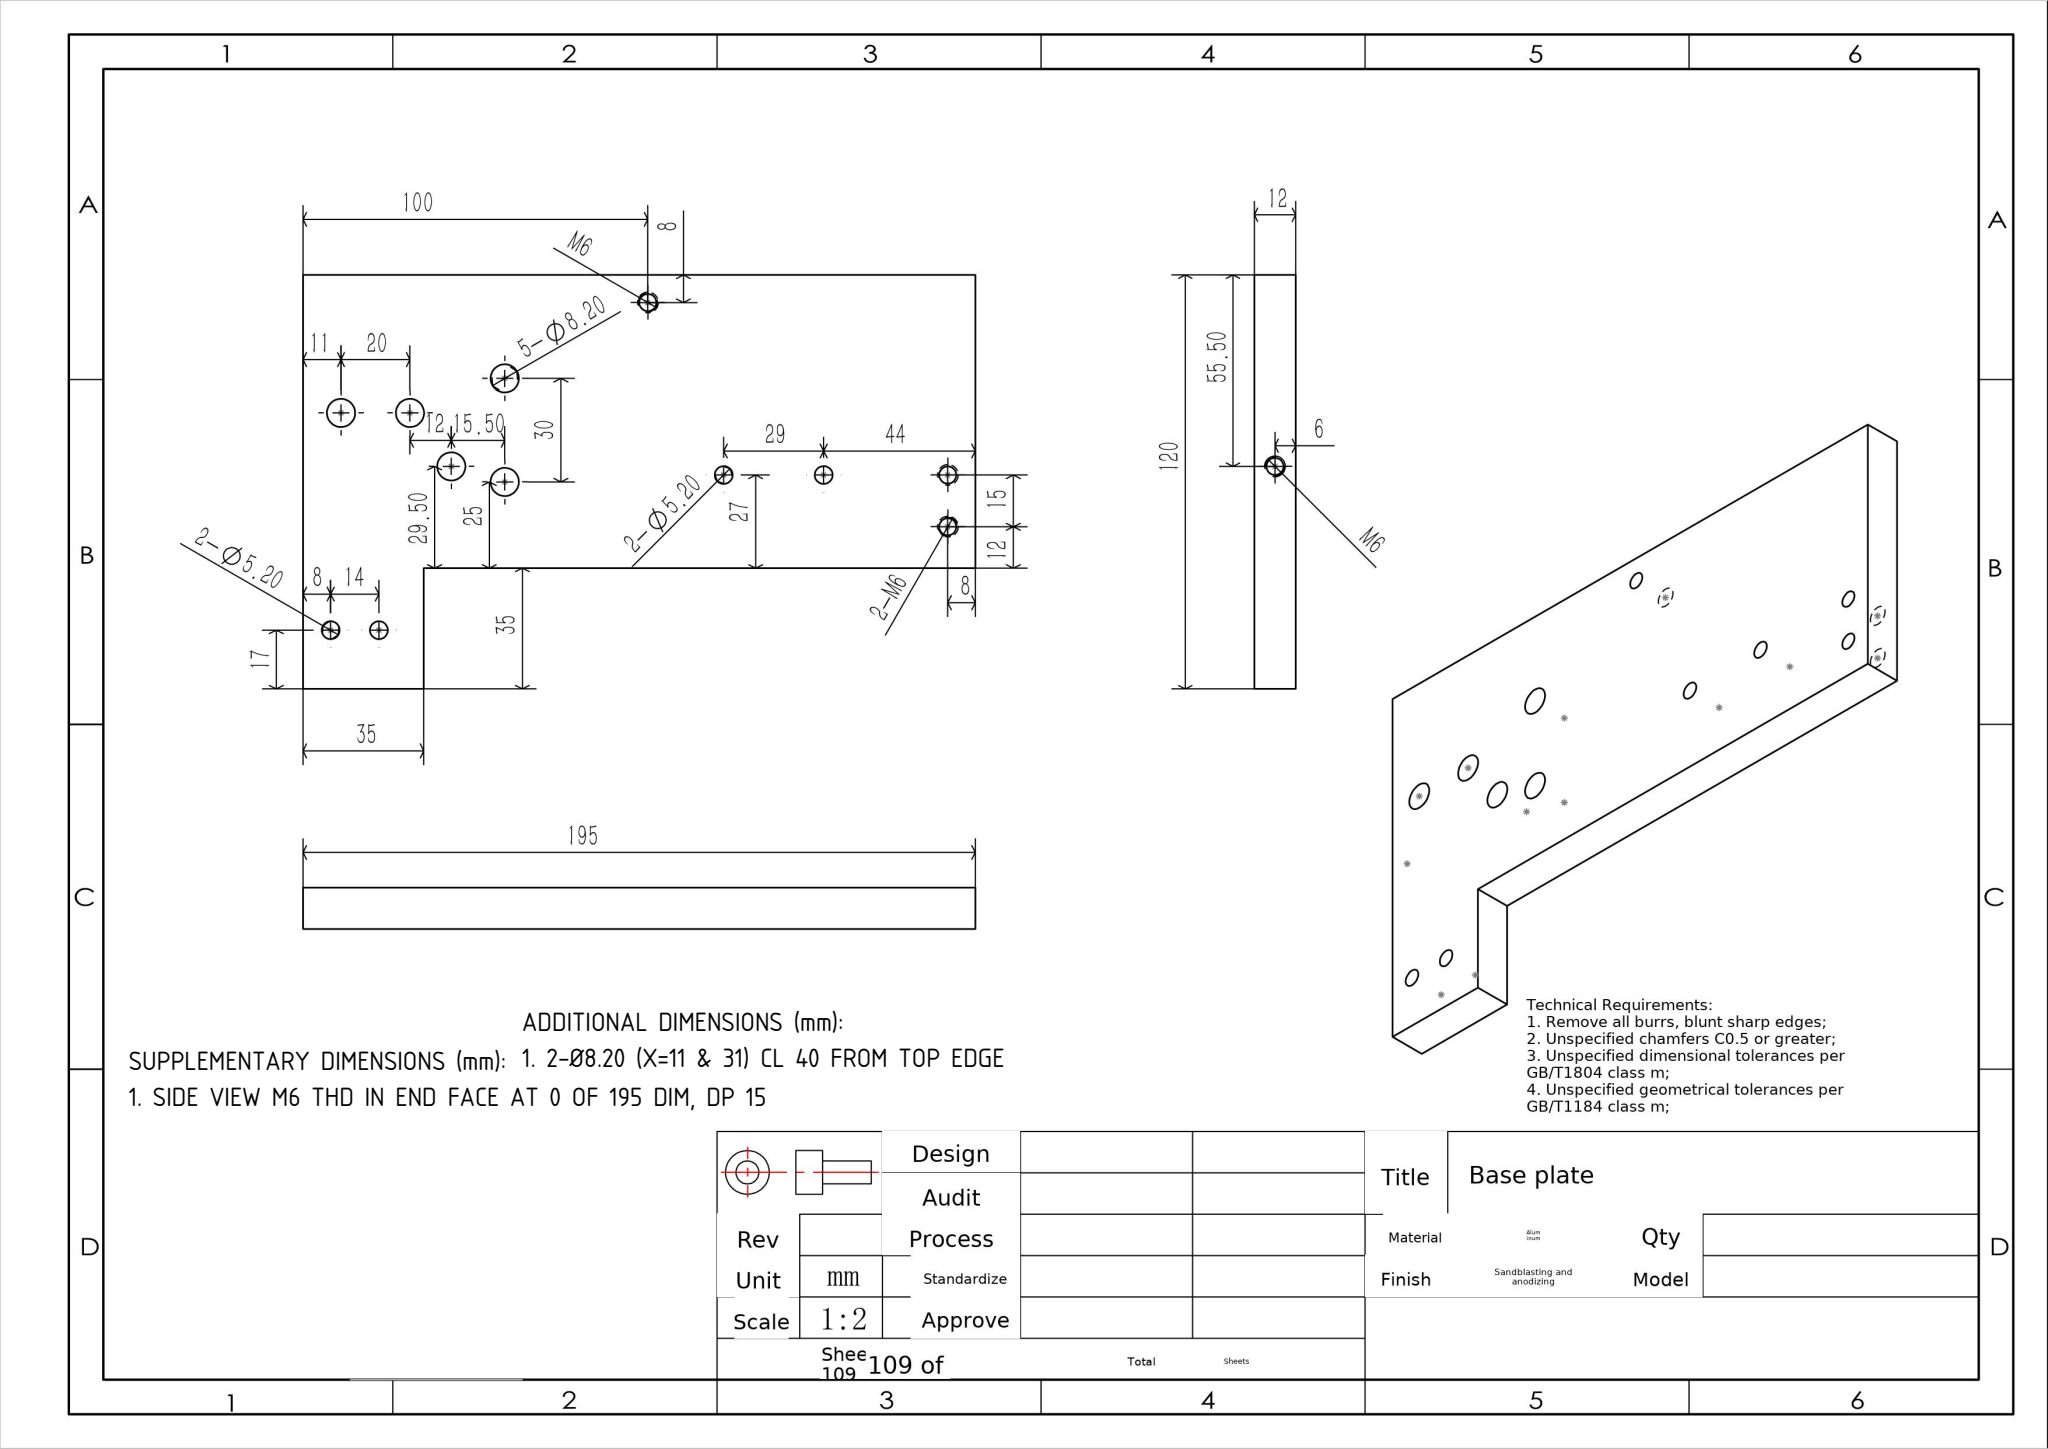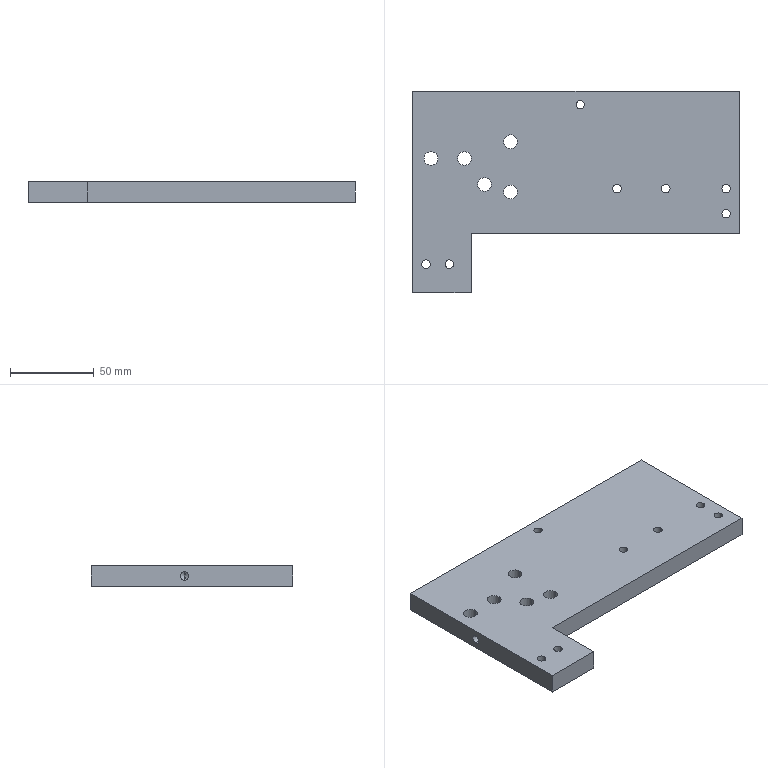Part | SolidWorks | mm | 1 solid | 36 faces | box 195 x 120 x 12 mm | volume 208401 mm3 | cylinder 26 | plane 8 | cone 2 | commonest cylinder face diameters 8.2 x10 5 x8 5.2 x8
build123d program:
from build123d import *

# Parameters (mm, degrees)
SKETCH1_W                      = 180
SKETCH1_H                      = 80
BOSS_EXTRUDE1_DEPTH            = 12
SKETCH2_W                      = 145
SKETCH2_H                      = 35
CUT_EXTRUDE1_DEPTH             = 12
F_5_2_5_2_DIAMETER_HOLE1_D     = 5.2
F_5_2_5_2_DIAMETER_HOLE1_DEPTH = 40
F_5_2_5_2_DIAMETER_HOLE1_TIP   = 1.562
F_5_2_5_2_DIAMETER_HOLE2_D     = 5.2
F_5_2_5_2_DIAMETER_HOLE2_DEPTH = 40
F_5_2_5_2_DIAMETER_HOLE2_TIP   = 1.562
F_8_2_8_2_DIAMETER_HOLE1_D     = 8.2
F_8_2_8_2_DIAMETER_HOLE1_DEPTH = 40
F_8_2_8_2_DIAMETER_HOLE1_TIP   = 2.464
M6_TAPPED_HOLE1_D              = 5
M6_TAPPED_HOLE1_DEPTH          = 15
M6_TAPPED_HOLE1_TIP            = 1.502
SKETCH14_W                     = 180
SKETCH14_H                     = 12
BOSS_EXTRUDE2_DEPTH            = 40
F_8_2_8_2_DIAMETER_HOLE2_D     = 8.2
F_8_2_8_2_DIAMETER_HOLE2_DEPTH = 40
F_8_2_8_2_DIAMETER_HOLE2_TIP   = 2.464
F_8_2_8_2_DIAMETER_HOLE3_D     = 8.2
F_8_2_8_2_DIAMETER_HOLE3_DEPTH = 40
F_8_2_8_2_DIAMETER_HOLE3_TIP   = 2.464
SKETCH19_W                     = 12
SKETCH19_H                     = 85
BOSS_EXTRUDE3_DEPTH            = 15
M6_TAPPED_HOLE2_D              = 5
M6_TAPPED_HOLE2_DEPTH          = 15
M6_TAPPED_HOLE2_TIP            = 1.502
M6_TAPPED_HOLE3_D              = 5
M6_TAPPED_HOLE3_DEPTH          = 15
M6_TAPPED_HOLE3_TIP            = 1.502


with BuildPart() as part:
    # Sketch1 → Boss-Extrude1 (new body)
    with BuildSketch(Plane.XY):
        with Locations((90, -40)):
            Rectangle(SKETCH1_W, SKETCH1_H)
    extrude(amount=BOSS_EXTRUDE1_DEPTH)

    # Sketch2 → Cut-Extrude1 (cut)
    with BuildSketch(Plane.XY.offset(12)):
        with Locations((107.5, -62.5)):
            Rectangle(SKETCH2_W, SKETCH2_H)
    extrude(amount=-CUT_EXTRUDE1_DEPTH, mode=Mode.SUBTRACT)

    # 5.2 _5.2_ Diameter Hole1
    with Locations(Plane(origin=(22, -63, 0), x_dir=(-1, 0, 0), z_dir=(0, 0, -1))):
        with Locations((0, 0), (14, 0)):
            Hole(F_5_2_5_2_DIAMETER_HOLE1_D / 2, depth=F_5_2_5_2_DIAMETER_HOLE1_DEPTH)
            with Locations((0, 0, -(F_5_2_5_2_DIAMETER_HOLE1_DEPTH + F_5_2_5_2_DIAMETER_HOLE1_TIP / 2))):  # 118° drill point
                Cone(0, F_5_2_5_2_DIAMETER_HOLE1_D / 2, F_5_2_5_2_DIAMETER_HOLE1_TIP, mode=Mode.SUBTRACT)

    # 5.2 _5.2_ Diameter Hole2
    with Locations(Plane(origin=(151, -18, 0), x_dir=(-1, 0, 0), z_dir=(0, 0, -1))):
        with Locations((0, 0), (29, 0)):
            Hole(F_5_2_5_2_DIAMETER_HOLE2_D / 2, depth=F_5_2_5_2_DIAMETER_HOLE2_DEPTH)
            with Locations((0, 0, -(F_5_2_5_2_DIAMETER_HOLE2_DEPTH + F_5_2_5_2_DIAMETER_HOLE2_TIP / 2))):  # 118° drill point
                Cone(0, F_5_2_5_2_DIAMETER_HOLE2_D / 2, F_5_2_5_2_DIAMETER_HOLE2_TIP, mode=Mode.SUBTRACT)

    # 8.2 _8.2_ Diameter Hole1
    with Locations(Plane(origin=(43, -15.5, 0), x_dir=(-1, 0, 0), z_dir=(0, 0, -1))):
        with Locations((0, 0)):
            Hole(F_8_2_8_2_DIAMETER_HOLE1_D / 2, depth=F_8_2_8_2_DIAMETER_HOLE1_DEPTH)
            with Locations((0, 0, -(F_8_2_8_2_DIAMETER_HOLE1_DEPTH + F_8_2_8_2_DIAMETER_HOLE1_TIP / 2))):  # 118° drill point
                Cone(0, F_8_2_8_2_DIAMETER_HOLE1_D / 2, F_8_2_8_2_DIAMETER_HOLE1_TIP, mode=Mode.SUBTRACT)

    # M6 Tapped Hole1
    with Locations(Plane(origin=(0, -15.5, 6), x_dir=(0, -1, 0), z_dir=(-1, 0, 0))):
        with Locations((0, 0)):
            Hole(M6_TAPPED_HOLE1_D / 2, depth=M6_TAPPED_HOLE1_DEPTH)
            with Locations((0, 0, -(M6_TAPPED_HOLE1_DEPTH + M6_TAPPED_HOLE1_TIP / 2))):  # 118° drill point
                Cone(0, M6_TAPPED_HOLE1_D / 2, M6_TAPPED_HOLE1_TIP, mode=Mode.SUBTRACT)

    # Sketch14 → Boss-Extrude2 (add)
    with BuildSketch(Plane(origin=(0, 0, 0), x_dir=(1, 0, 0), z_dir=(0, 1, 0))):
        with Locations((90, -6)):
            Rectangle(SKETCH14_W, SKETCH14_H)
    extrude(amount=BOSS_EXTRUDE2_DEPTH)

    # 8.2 _8.2_ Diameter Hole2
    with Locations(Plane(origin=(58.5, -20, 0), x_dir=(-1, 0, 0), z_dir=(0, 0, -1))):
        with Locations((0, 0), (0, 30)):
            Hole(F_8_2_8_2_DIAMETER_HOLE2_D / 2, depth=F_8_2_8_2_DIAMETER_HOLE2_DEPTH)
            with Locations((0, 0, -(F_8_2_8_2_DIAMETER_HOLE2_DEPTH + F_8_2_8_2_DIAMETER_HOLE2_TIP / 2))):  # 118° drill point
                Cone(0, F_8_2_8_2_DIAMETER_HOLE2_D / 2, F_8_2_8_2_DIAMETER_HOLE2_TIP, mode=Mode.SUBTRACT)

    # 8.2 _8.2_ Diameter Hole3
    with Locations(Plane(origin=(11, 0, 12), x_dir=(1, 0, 0), z_dir=(0, 0, 1))):
        with Locations((0, 0), (20, 0)):
            Hole(F_8_2_8_2_DIAMETER_HOLE3_D / 2, depth=F_8_2_8_2_DIAMETER_HOLE3_DEPTH)
            with Locations((0, 0, -(F_8_2_8_2_DIAMETER_HOLE3_DEPTH + F_8_2_8_2_DIAMETER_HOLE3_TIP / 2))):  # 118° drill point
                Cone(0, F_8_2_8_2_DIAMETER_HOLE3_D / 2, F_8_2_8_2_DIAMETER_HOLE3_TIP, mode=Mode.SUBTRACT)

    # Sketch19 → Boss-Extrude3 (add)
    with BuildSketch(Plane(origin=(180, 0, 0), x_dir=(0, 0, -1), z_dir=(1, 0, 0))):
        with Locations((-6, -2.5)):
            Rectangle(SKETCH19_W, SKETCH19_H)
    extrude(amount=BOSS_EXTRUDE3_DEPTH)

    # M6 Tapped Hole2
    with Locations(Plane(origin=(187, -18, 0), x_dir=(-1, 0, 0), z_dir=(0, 0, -1))):
        with Locations((0, 0), (0, -15)):
            Hole(M6_TAPPED_HOLE2_D / 2, depth=M6_TAPPED_HOLE2_DEPTH)
            with Locations((0, 0, -(M6_TAPPED_HOLE2_DEPTH + M6_TAPPED_HOLE2_TIP / 2))):  # 118° drill point
                Cone(0, M6_TAPPED_HOLE2_D / 2, M6_TAPPED_HOLE2_TIP, mode=Mode.SUBTRACT)

    # M6 Tapped Hole3
    with Locations(Plane(origin=(100, 32, 0), x_dir=(-1, 0, 0), z_dir=(0, 0, -1))):
        with Locations((0, 0)):
            Hole(M6_TAPPED_HOLE3_D / 2, depth=M6_TAPPED_HOLE3_DEPTH)
            with Locations((0, 0, -(M6_TAPPED_HOLE3_DEPTH + M6_TAPPED_HOLE3_TIP / 2))):  # 118° drill point
                Cone(0, M6_TAPPED_HOLE3_D / 2, M6_TAPPED_HOLE3_TIP, mode=Mode.SUBTRACT)


solid = part.part